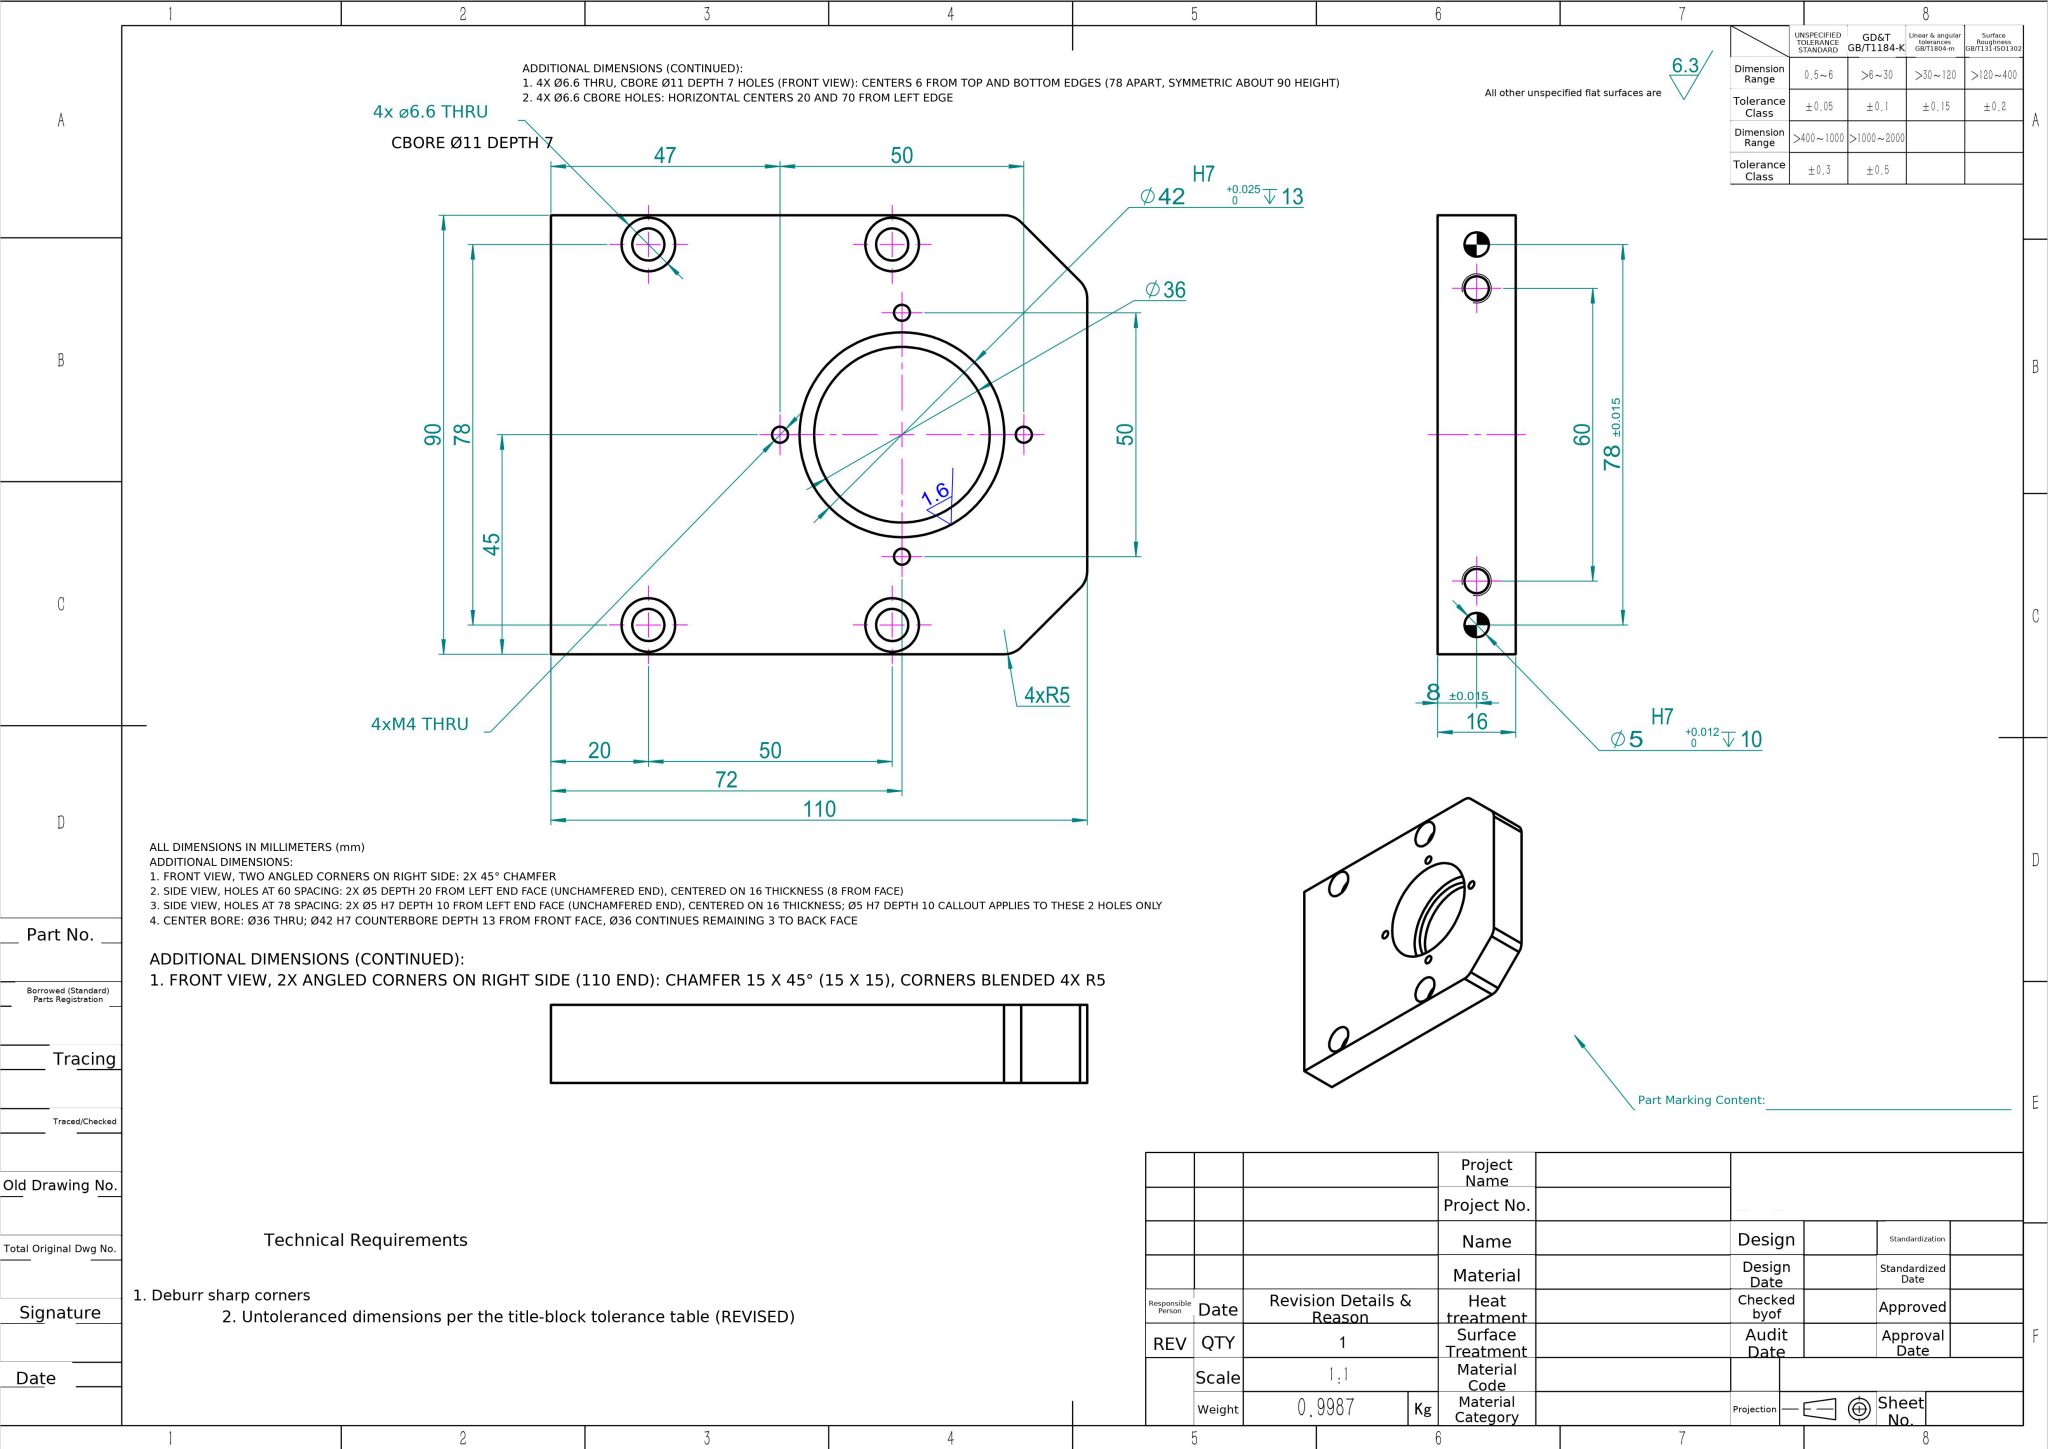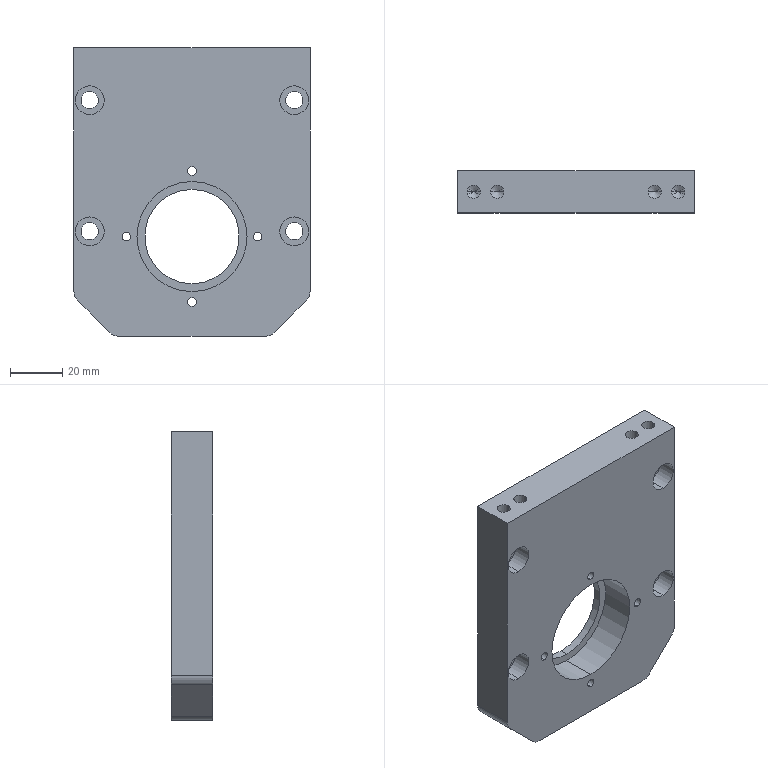Part | NX | mm | 1 solid | 61 faces | box 90 x 16 x 110 mm | volume 128044 mm3 | cylinder 40 | plane 13 | cone 8 | commonest cylinder face diameters 3.3 x8 5 x8 11 x8 6.6 x8 10 x4 42 x2 36 x2